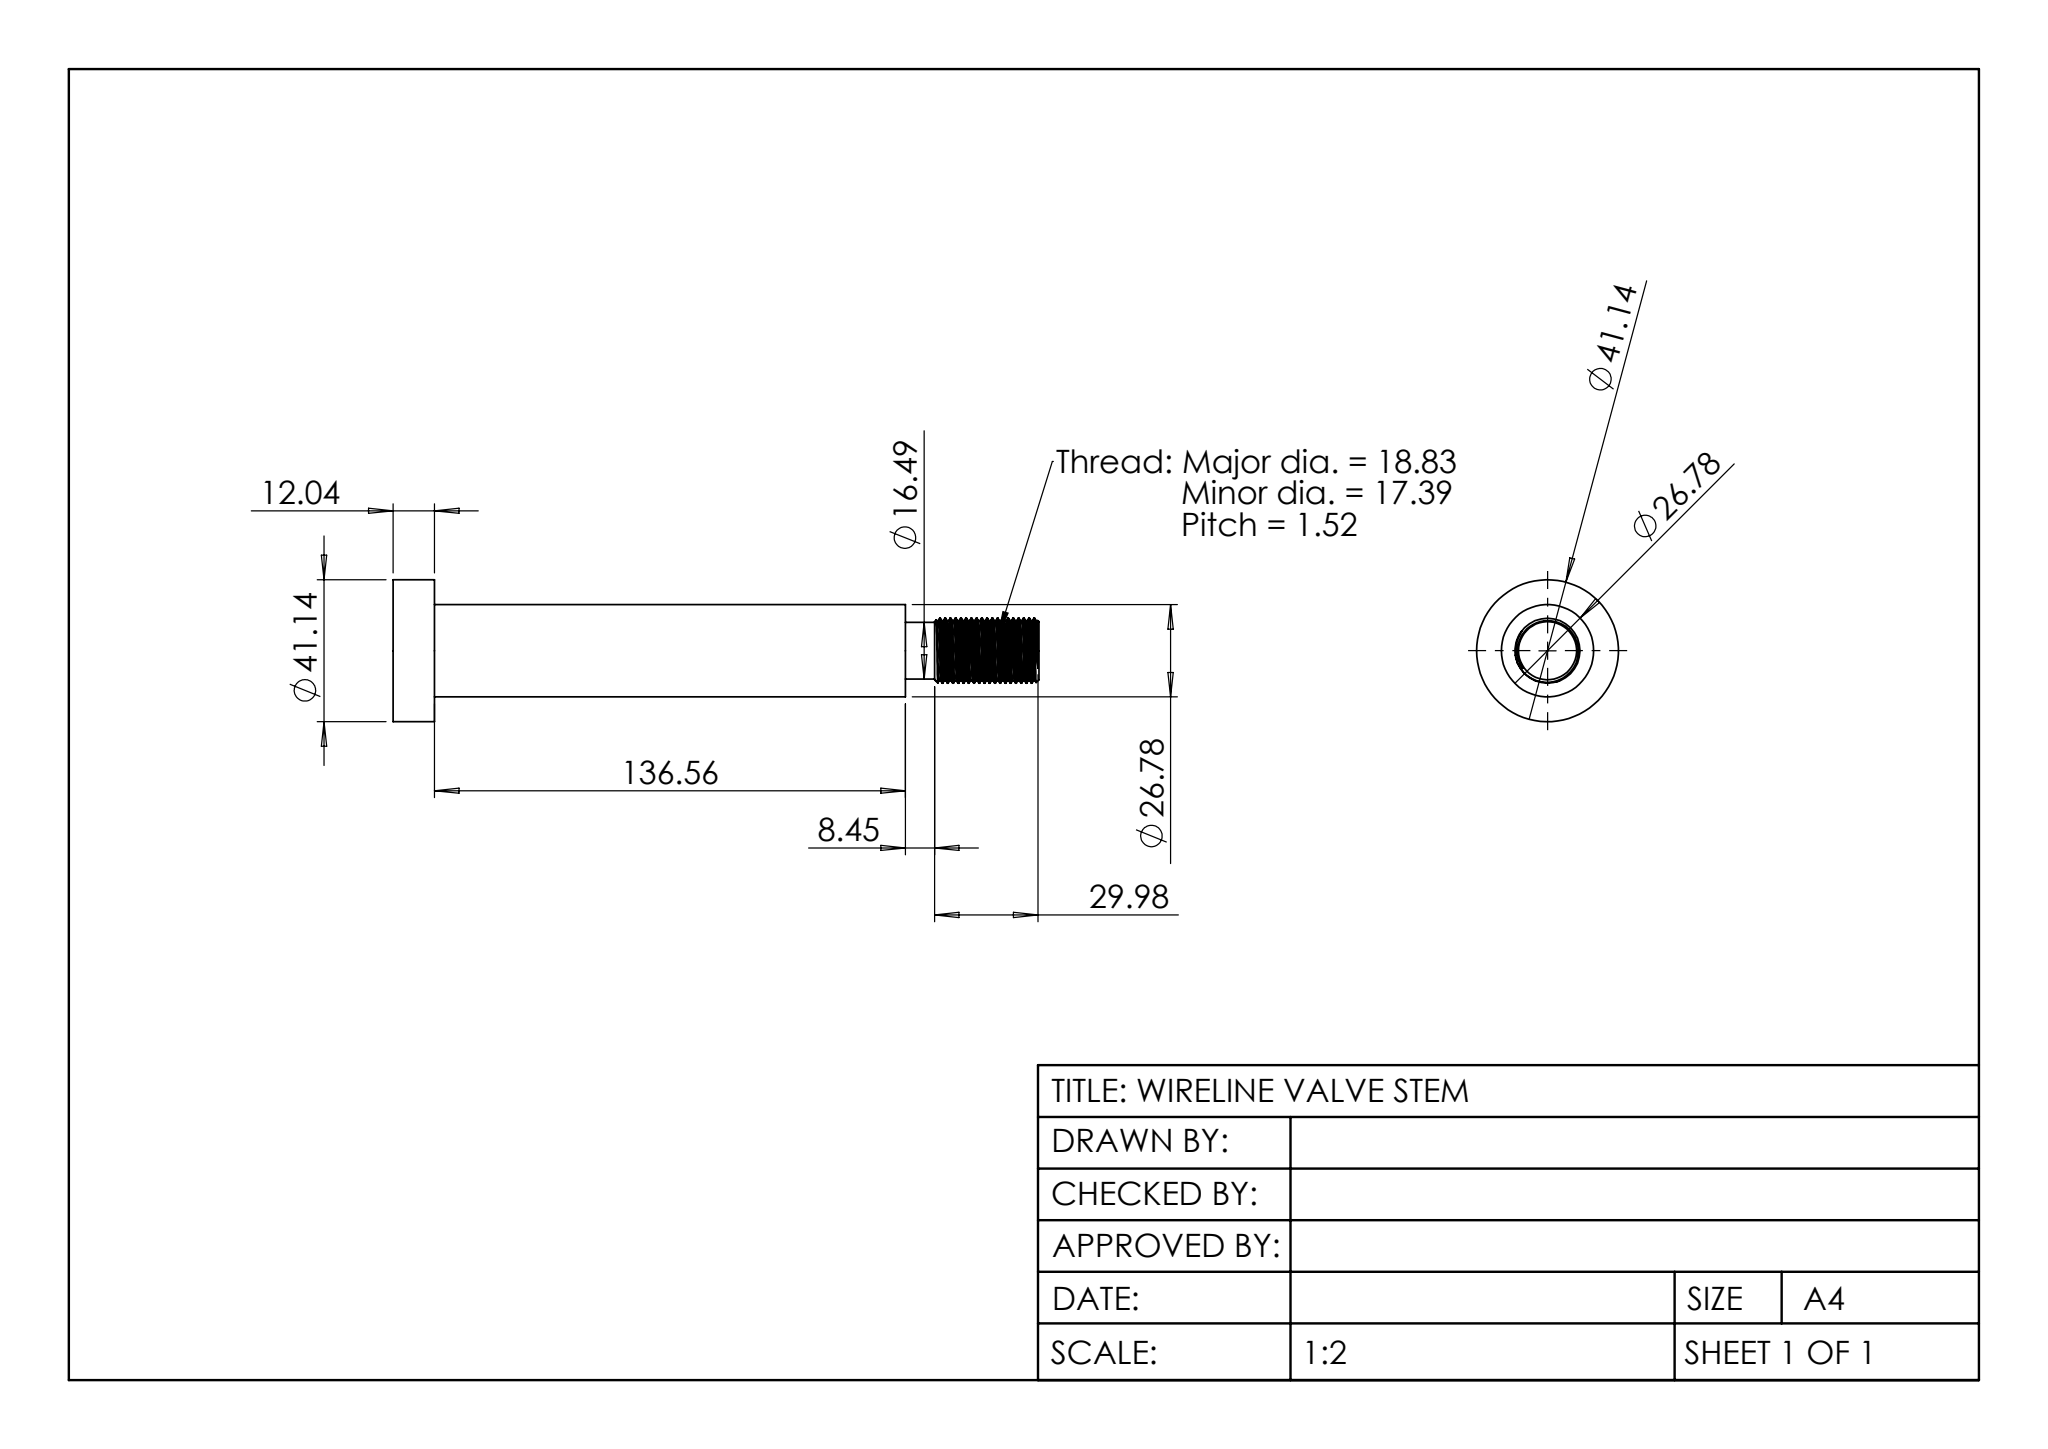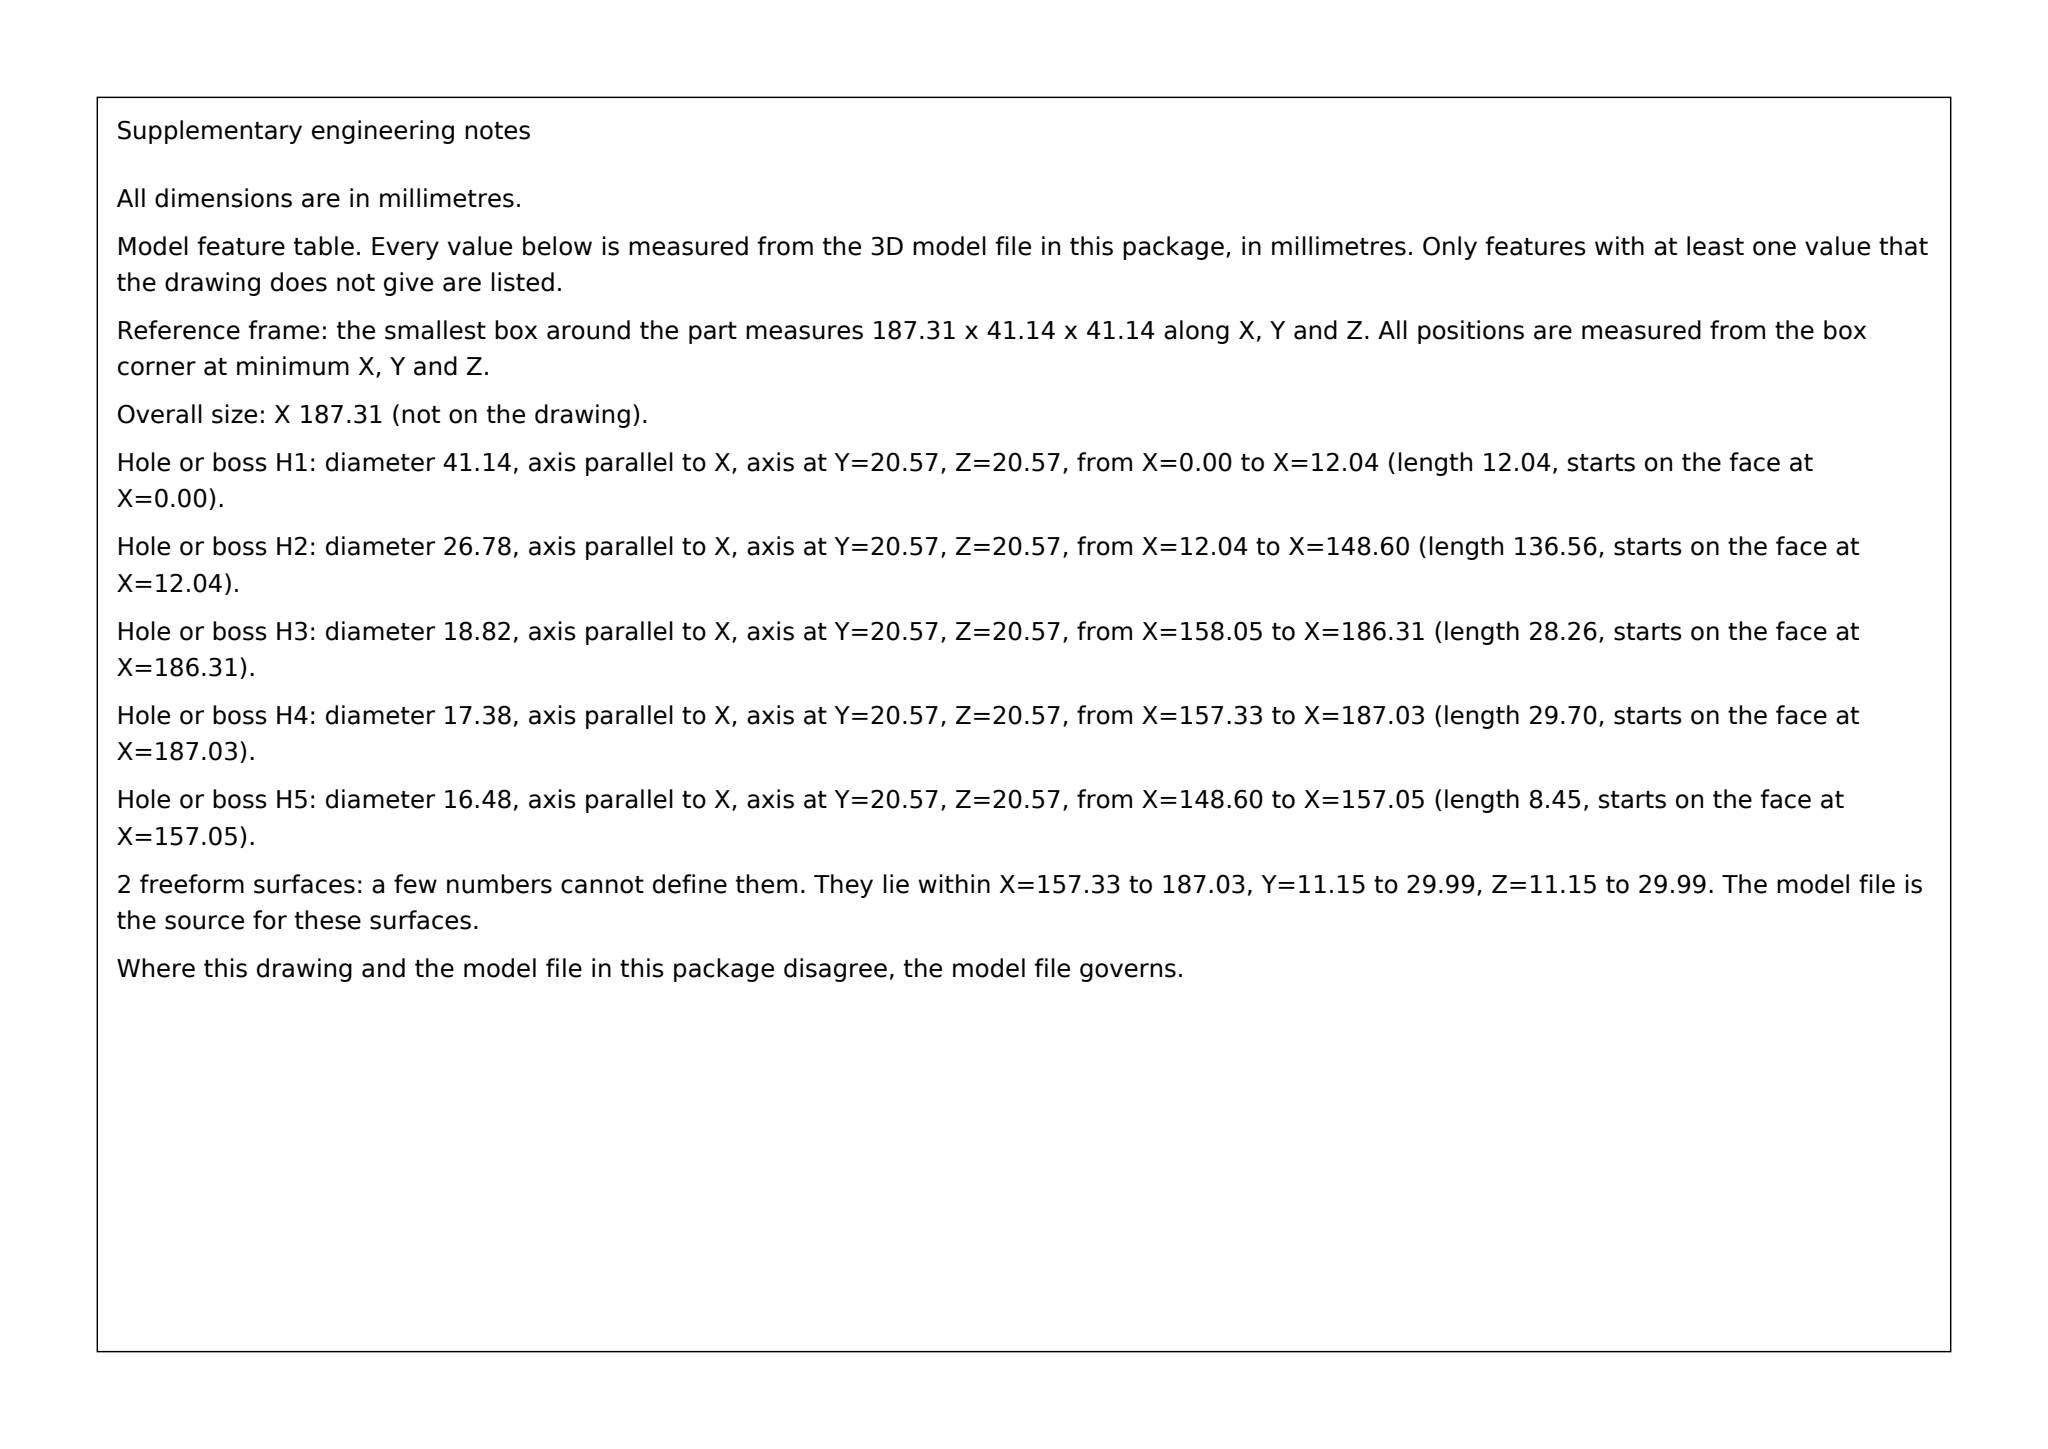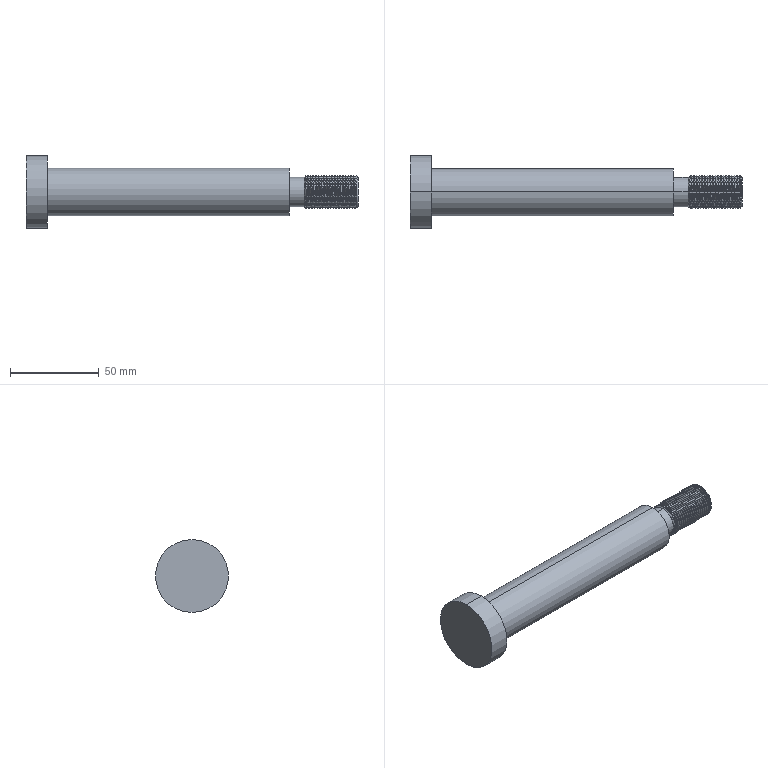Part | SolidWorks | mm | 1 solid | 98 faces | box 187.31 x 41.14 x 41.14 mm | volume 102381 mm3 | cylinder 86 | cone 5 | plane 5 | spline 2 | commonest cylinder face diameters 17.39 x41 18.83 x39 16.49 x2 26.78 x2 41.14 x2